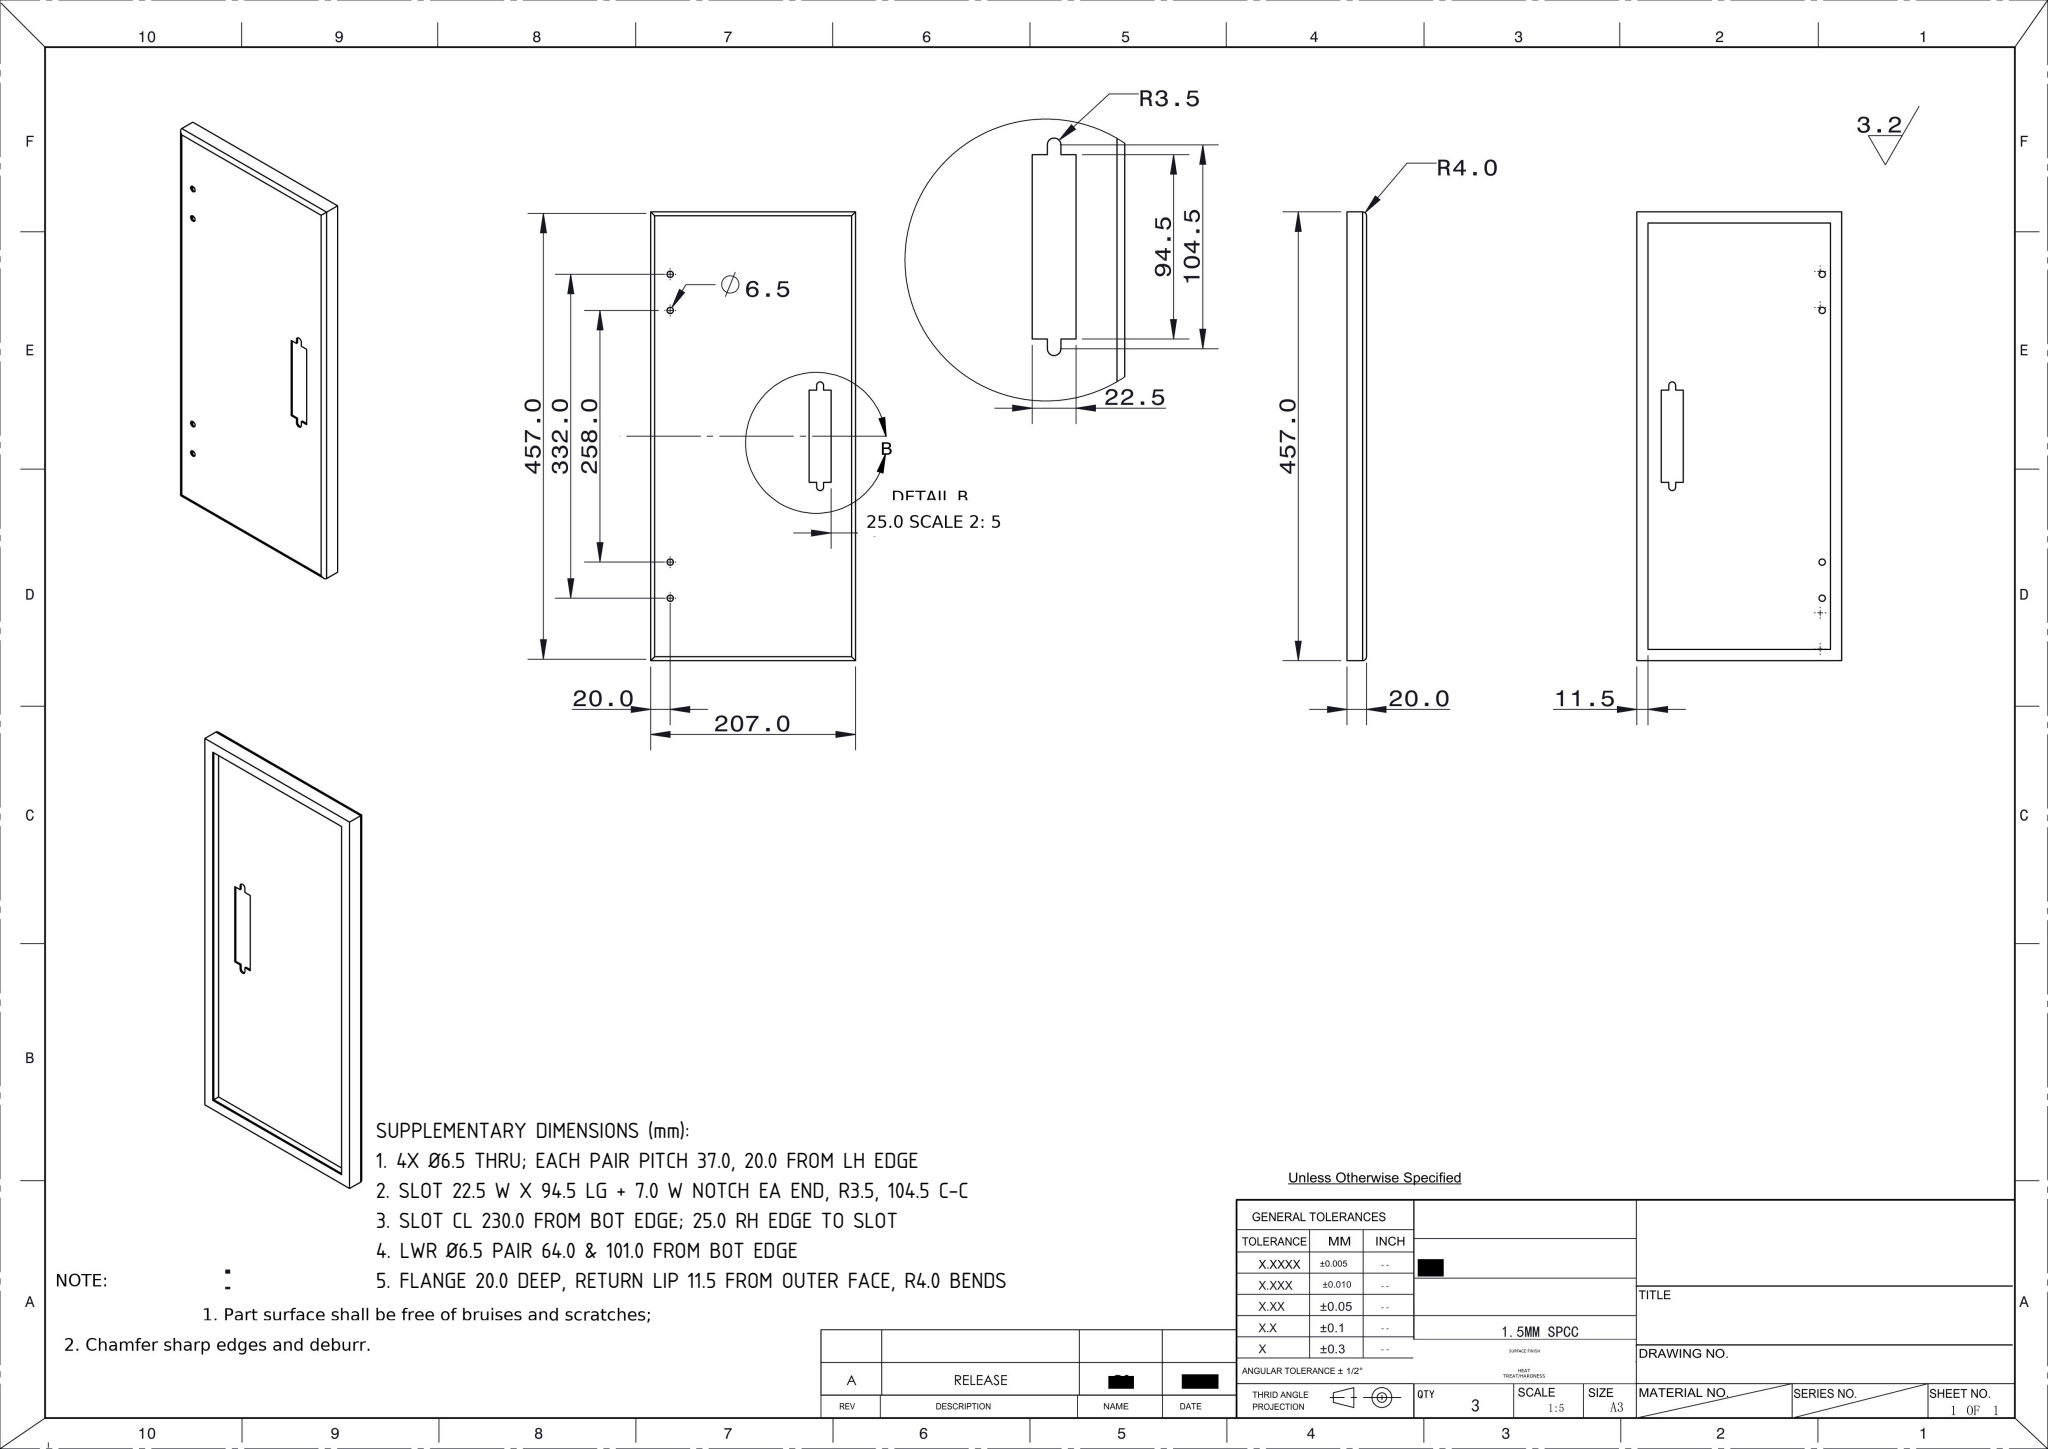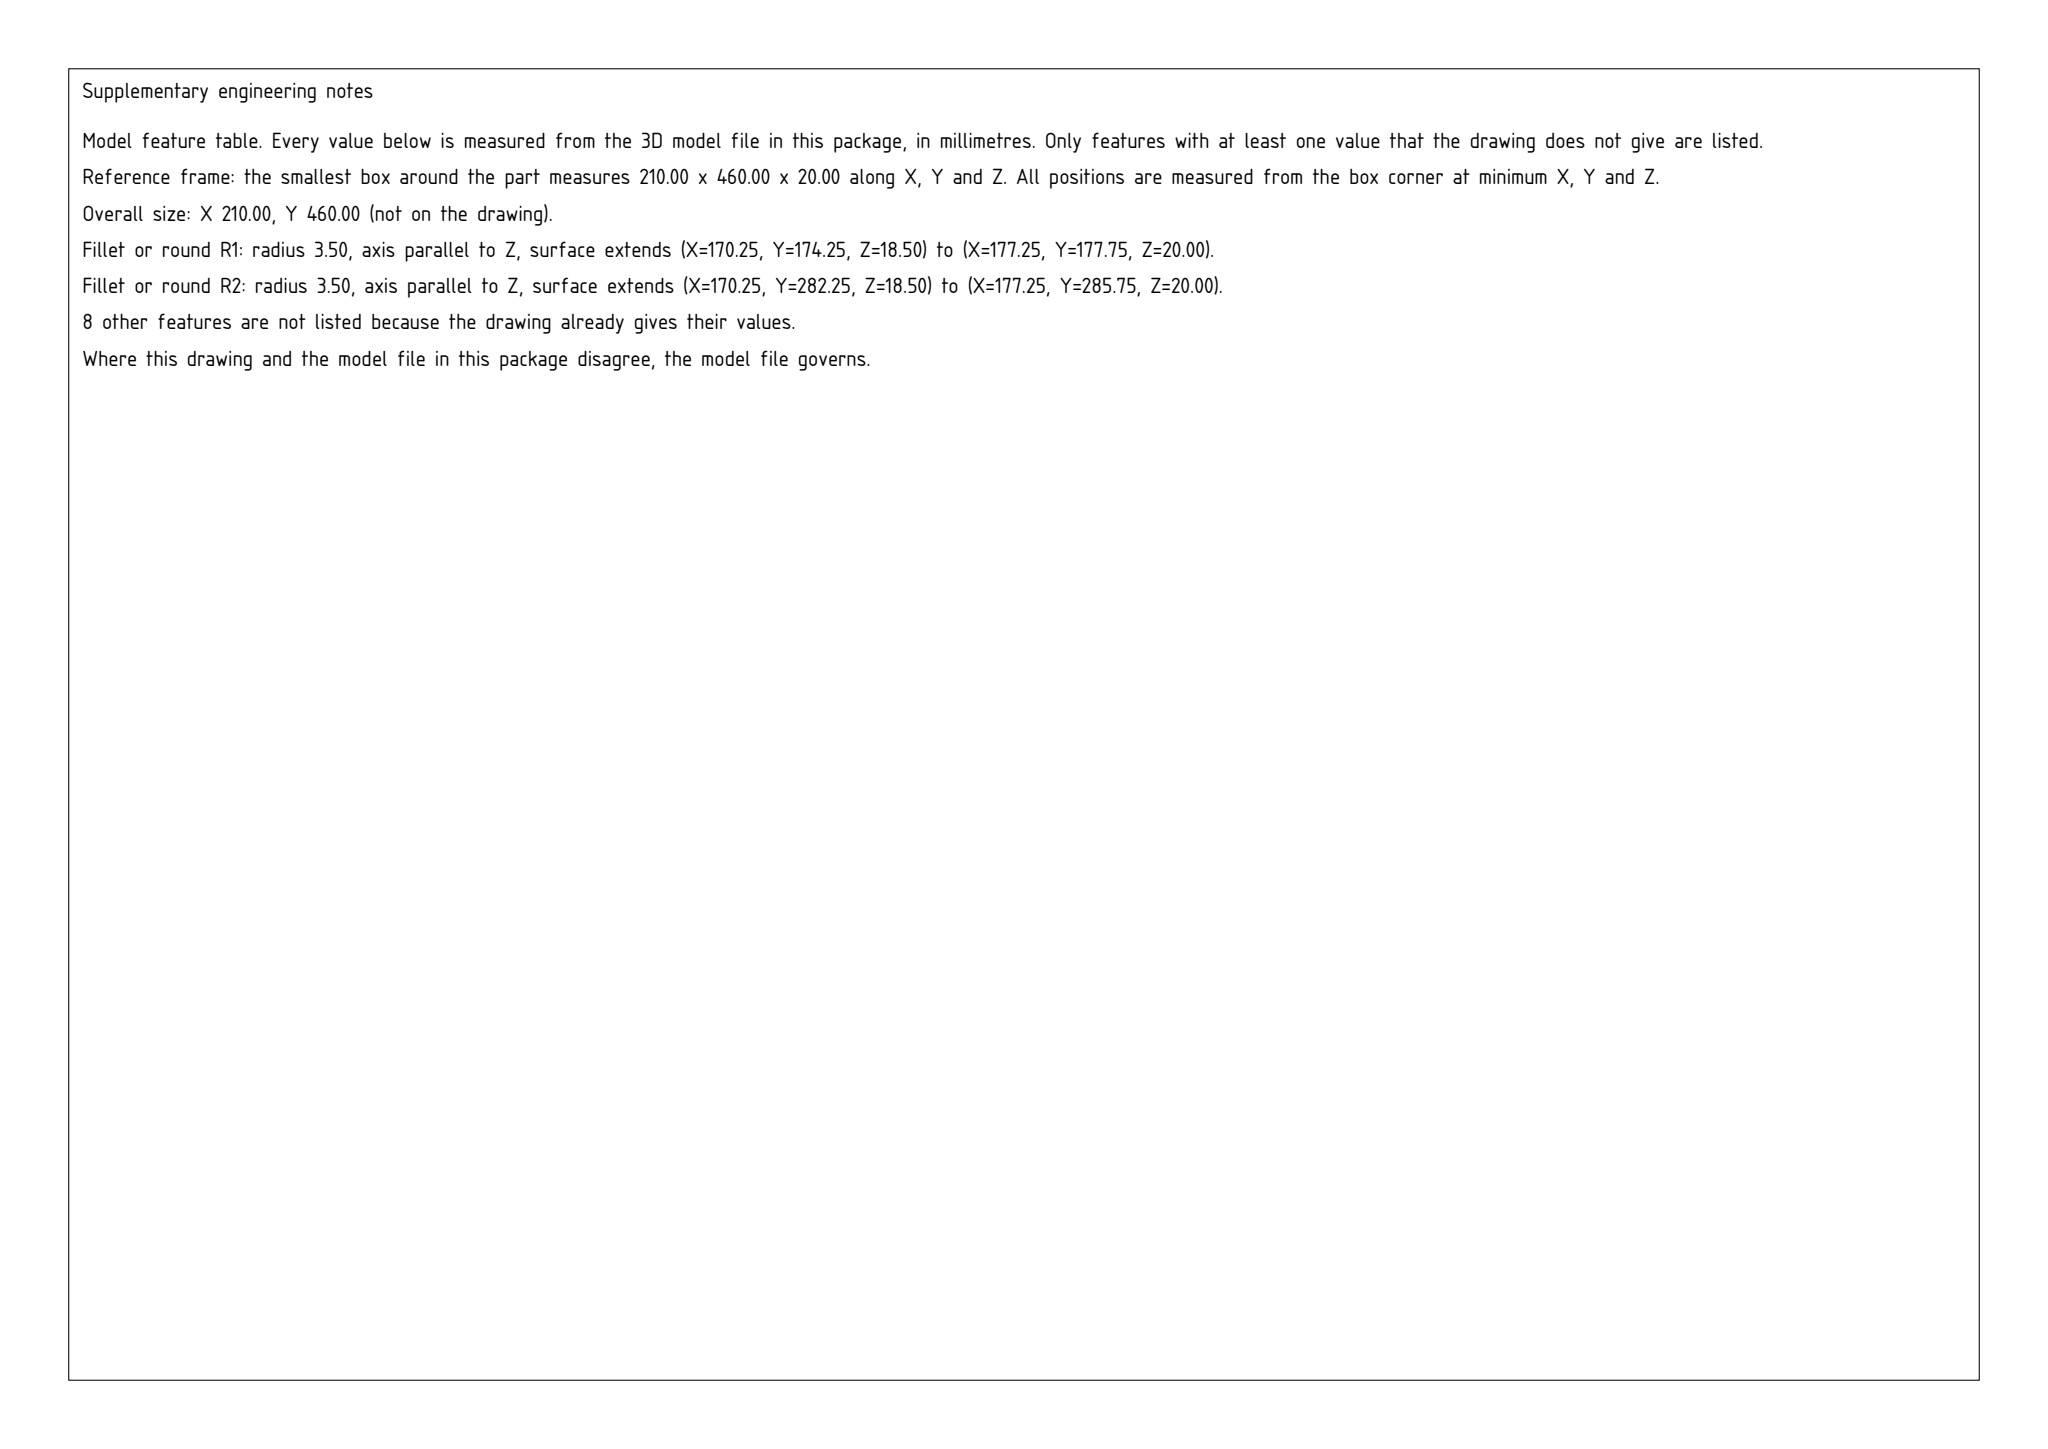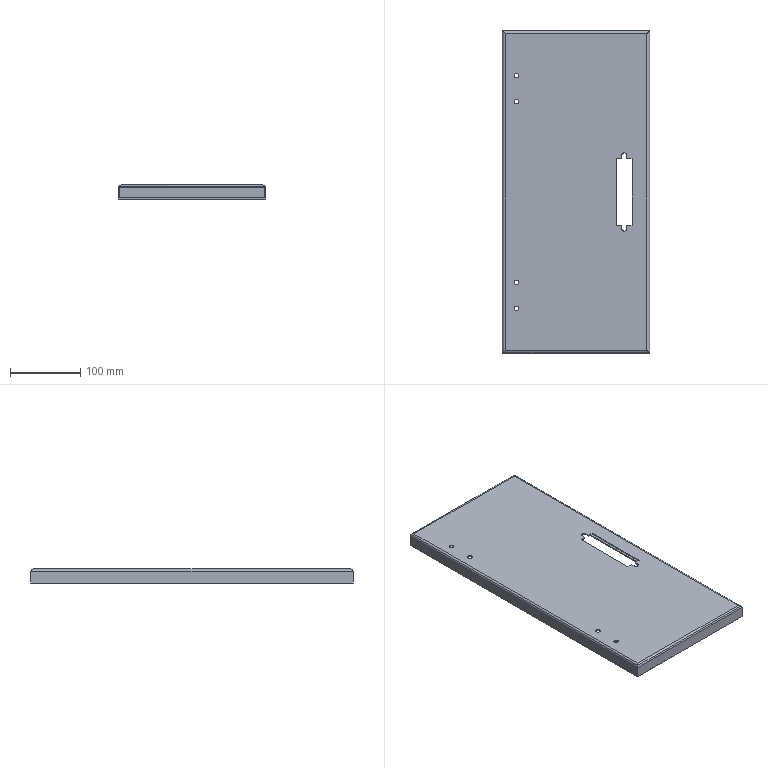Part | SolidWorks | mm | 1 solid | 40 faces | box 210 x 460 x 20 mm | volume 193111 mm3 | plane 26 | cylinder 14 | commonest cylinder face diameters 6.5 x8 8 x4 7 x2
build123d program:
from build123d import *

# Parameters (mm, degrees)
SKETCH1_W                  = 210
SKETCH1_H                  = 460
BOSS_EXTRUDE1_DEPTH        = 20
SHELL1_T                   = -1.5
SKETCH2_W                  = 207
SKETCH2_H                  = 1.5
BOSS_EXTRUDE2_DEPTH        = 10
SKETCH3_W                  = 1.5
SKETCH3_H                  = 447
BOSS_EXTRUDE3_DEPTH        = 10
SKETCH5_W                  = 197
SKETCH5_H                  = 1.5
BOSS_EXTRUDE4_DEPTH        = 10
SKETCH6_W                  = 1.5
SKETCH6_H                  = 437
BOSS_EXTRUDE5_DEPTH        = 10
FILLET2_R                  = 4
F_6_5_6_5_DIAMETER_HOLE1_D = 6.5
CUT_EXTRUDE1_DEPTH         = 10


with BuildPart() as part:
    # Sketch1 → Boss-Extrude1 (new body)
    with BuildSketch(Plane.XY):
        with Locations((-13752.87, 4762.21)):
            Rectangle(SKETCH1_W, SKETCH1_H)
    extrude(amount=BOSS_EXTRUDE1_DEPTH)

    # Shell1
    shell1_openings = [part.faces().sort_by_distance(p)[0] for p in [
        (-13752.87, 4762.21, 0),
    ]]
    offset(amount=SHELL1_T, openings=shell1_openings, kind=Kind.INTERSECTION)

    # Sketch2 → Boss-Extrude2 (add)
    with BuildSketch(Plane(origin=(0, 4533.71, 0), x_dir=(-1, 0, 0), z_dir=(0, 1, 0))):
        with Locations((13752.87, 0.75)):
            Rectangle(SKETCH2_W, SKETCH2_H)
    extrude(amount=BOSS_EXTRUDE2_DEPTH)

    # Sketch3 → Boss-Extrude3 (add)
    with BuildSketch(Plane.ZY.offset(13649.37)):
        with Locations((0.75, 4767.21)):
            Rectangle(SKETCH3_W, SKETCH3_H)
    extrude(amount=BOSS_EXTRUDE3_DEPTH)

    # Sketch5 → Boss-Extrude4 (add)
    with BuildSketch(Plane(origin=(0, 4990.71, 0), x_dir=(-1, 0, 0), z_dir=(0, -1, 0))):
        with Locations((13757.87, -0.75)):
            Rectangle(SKETCH5_W, SKETCH5_H)
    extrude(amount=BOSS_EXTRUDE4_DEPTH)

    # Sketch6 → Boss-Extrude5 (add)
    with BuildSketch(Plane(origin=(-13856.37, 0, 0), x_dir=(0, 0, -1), z_dir=(1, 0, 0))):
        with Locations((-0.75, 4762.21)):
            Rectangle(SKETCH6_W, SKETCH6_H)
    extrude(amount=BOSS_EXTRUDE5_DEPTH)

    # Fillet2
    fillet2_edges = [part.edges().sort_by_distance(p)[0] for p in [
        (-13857.87, 4762.21, 20),
        (-13752.87, 4532.21, 20),
        (-13647.87, 4762.21, 20),
        (-13752.87, 4992.21, 20),
    ]]
    fillet(fillet2_edges, radius=FILLET2_R)

    # 6.5 _6.5_ Diameter Hole1 (through all)
    with Locations(Plane.XY.offset(20)):
        with Locations((-13837.87, 4928.21), (-13837.87, 4891.21), (-13837.87, 4633.21), (-13837.87, 4596.21)):
            Hole(F_6_5_6_5_DIAMETER_HOLE1_D / 2)

    # Sketch8 → Cut-Extrude1 (cut)
    with BuildSketch(Plane.XY.offset(20)):
        with BuildLine():
            Line((-13695.37, 4714.96), (-13695.37, 4809.46))
            Line((-13695.37, 4809.46), (-13687.62, 4809.46))
            Line((-13687.62, 4809.46), (-13687.62, 4814.46))
            ThreePointArc((-13687.62, 4814.46), (-13684.12, 4817.96), (-13680.62, 4814.46))
            Line((-13680.62, 4814.46), (-13680.62, 4809.46))
            Line((-13680.62, 4809.46), (-13672.87, 4809.46))
            Line((-13672.87, 4809.46), (-13672.87, 4714.96))
            Line((-13672.87, 4714.96), (-13680.62, 4714.96))
            Line((-13680.62, 4714.96), (-13680.62, 4709.96))
            ThreePointArc((-13680.62, 4709.96), (-13684.12, 4706.46), (-13687.62, 4709.96))
            Line((-13687.62, 4709.96), (-13687.62, 4714.96))
            Line((-13687.62, 4714.96), (-13695.37, 4714.96))
        make_face()
    extrude(amount=-CUT_EXTRUDE1_DEPTH, mode=Mode.SUBTRACT)


solid = part.part